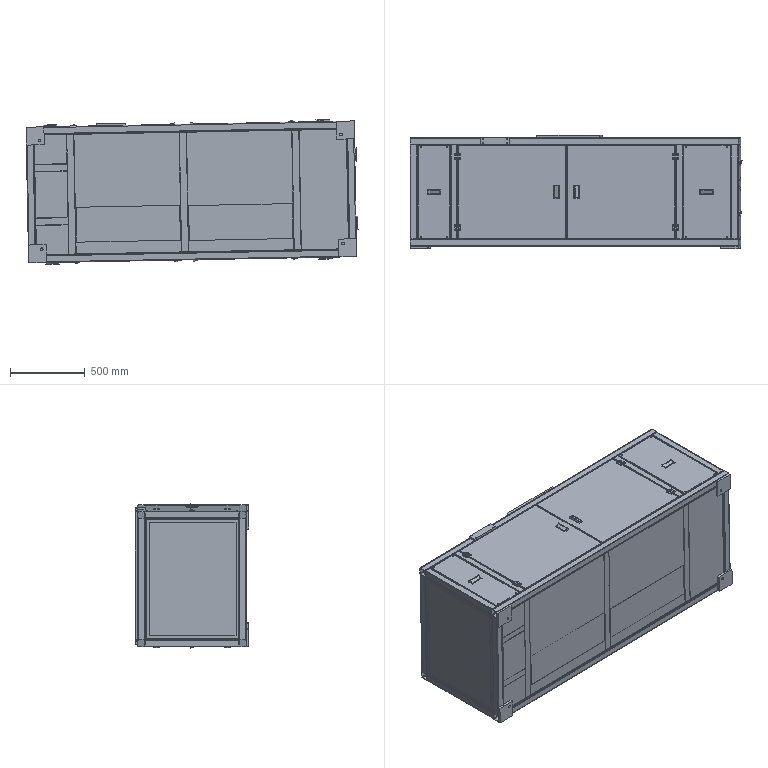Assembly | SolidWorks | mm | 44 component files | 133 solids | 3777 faces | box 2225.49 x 760 x 970.37 mm | volume 42957935 mm3 | plane 2257 | cylinder 1328 | cone 192 | commonest cylinder face diameters 6 x200 10 x144 7 x122 2 x120 5 x104 4.2 x100 4 x88 11 x72
Bill of materials:
01Frame | 1 | A3 Steel | Elongated rectangular open frame built from square-section members, with corner blocks, intermediate vertical posts and cross members, one long side covered by a flat panel, and an internal partition panel near one end.
02FrameEndPlate1 | 2 | A3 Steel | Rectangular tray-like cover plate with shallow turned-down edge flanges, one central rectangular cutout and four corner holes.
03FrameEndPlate2 | 2 | A3 Steel | Long, narrow rectangular cover plate with shallow turned-down edge flanges, one central rectangular cutout and four corner holes.
04FrameEndPlate3 | 2 | A3 Steel | Tall rectangular flat panel with a shallow edge return, two vertically aligned rectangular slots on the centerline and small holes near the four corners.
05FrameEndPlate4 | 1 | A3 Steel | Rectangular flat panel with a shallow edge return, two vertically aligned rectangular slots on the centerline and small holes near the four corners. It is wider than the similar slotted panel.
09Panel2 | 1 | A3 Steel | Flat rectangular plate with a large rectangular window that has rounded corners, plus many small holes in clusters above and below the window and along the edges.
11BottomDoor | 2 | A3 Steel | Large, nearly square flat panel with a shallow perimeter flange, one off-center rectangular slot near an edge and a few small holes near two corners.
12TopPostMountingPlateSpacer | 2 | A3 Steel | Solid rectangular bar or block with two round through-holes passing through its narrow side face.
13TopPostMountingPlate | 1 | A3 Steel | Thick rectangular plate with two parallel columns of evenly spaced round holes and four elongated slots near the corners.
15BrushPlateThickInnerFrameOneOutOfTwo | 1 | A3 Steel | Rectangular frame plate with rounded outer corners, a large central opening with stepped notches, small mounting holes around the perimeter, and stepped raised rails along the inner edges.
16MeshPlateOneOutOfTwo | 1 | A3 Steel | Thin flat sheet plate with rounded corners, four long parallel slots, four larger corner holes and several small edge holes.
17DustCollectionHopper | 2 | A3 Steel | Long formed sheet channel panel: a flat face with a top return flange and curled hook-shaped flanges at both ends.
22DragChainMountingPlate | 1 | A3 Steel | Long, slender straight channel with a C-shaped cross-section and rounded bends, with small holes near both ends and at mid-length.
23BottomDoor2 | 2 | A3 Steel | Large, thin, nearly square panel with shallow bent-down edge flanges, one rectangular through-cutout near one edge, and small holes near two corners.
40X40AluminumAlloyHinge | 8 | A3 Steel | Square flat plate with four through-holes, one near each corner, and a cylindrical (rounded) rib on the underside running across the plate.
93X35EmbeddedHandleSlot87X30.5 | 14 | A3 Steel | Elongated prismatic block with a wedge-shaped (sloped) top on a narrower rectangular base, with a shallow L-shaped groove or recess on the sloped face.
PowerDistributionCabinet | 1 | A3 Steel | Plain solid rectangular block (cuboid) with no visible holes, cutouts or other features.
Mates:
1. coincident | 15BrushPlateThickInnerFrameOneOutOfTwo-1 face at (111.137, -1638.022, 1897.203) dir (0, -1, 0) | 16MeshPlateOneOutOfTwo-1 face at (104.662, -1638.022, 2237.141) dir (0, 1, 0)
2. coincident | 09Panel2-1 face at (76.81, -1621.522, 1861.543) dir (0, 1, 0) | 15BrushPlateThickInnerFrameOneOutOfTwo-1 face at (368.947, -1621.522, 2277.182) dir (0, -1, 0)
3. coincident | 09Panel2-1 face at (77.095, -1621.522, 1846.545) dir (-0.01904, 0, 0.9998) | 15BrushPlateThickInnerFrameOneOutOfTwo-1 face at (77.095, -1621.522, 1846.545) dir (0.01904, 0, -0.9998)
4. coincident | 09Panel2-1 face at (61.812, -1621.522, 1861.257) dir (0.9998, 0, 0.01904) | 15BrushPlateThickInnerFrameOneOutOfTwo-1 face at (61.812, -1621.522, 1861.257) dir (-0.9998, 0, -0.01904)
5. coincident | 11BottomDoor-1 face at (-158.243, -1995.522, 2387.162) dir (-0.01904, 0, 0.9998) | 93X35EmbeddedHandleSlot87X30.5-18 face at (157.2, -2041.272, 2393.17) dir (0.01904, 0, -0.9998)
6. coincident | 11BottomDoor-1 edge at (124.706, -1952.022, 2392.551) dir (0, -1, 0) | 93X35EmbeddedHandleSlot87X30.5-18 face at (124.82, -1952.022, 2386.552) dir (-0.9998, 0, -0.01904)
7. coincident | 13TopPostMountingPlate-1 plane at (1160.151, -1828.022, 2090.216) dir (0.9998, 0, 0.01904) | 12TopPostMountingPlateSpacer-1 plane at (1158.199, -1865.522, 2192.697) dir (0.9998, 0, 0.01904)
8. coincident | 01Frame-1 face at (257.063, -1995.522, 2375.069) dir (-0.01904, 0, 0.9998) | 02FrameEndPlate1-1 face at (1146.901, -1995.522, 2392.018) dir (0.01904, 0, -0.9998)
9. coincident | 01Frame-1 face at (273.631, -1995.522, 1505.226) dir (0.01904, 0, -0.9998) | 02FrameEndPlate1-2 face at (1163.47, -1995.522, 1522.176) dir (-0.01904, 0, 0.9998)
10. concentric | 01Frame-1 face at (1025.995, -2297.522, 1519.557) dir (0.01904, 0, -0.9998) r 2.5 | 02FrameEndPlate1-2 face at (1026.376, -2297.522, 1499.561) dir (0.01904, 0, -0.9998) r 3.5
11. coincident | 01Frame-1 face at (257.063, -1995.522, 2375.069) dir (-0.01904, 0, 0.9998) | 03FrameEndPlate2-1 face at (-682.767, -1995.522, 2357.167) dir (0.01904, 0, -0.9998)
12. concentric | 01Frame-1 face at (-770.251, -1693.522, 2355.501) dir (-0.01904, 0, 0.9998) r 2.5 | 03FrameEndPlate2-1 face at (-770.632, -1693.522, 2375.497) dir (-0.01904, 0, 0.9998) r 3.5
13. concentric | 01Frame-1 face at (-595.283, -2297.522, 2358.833) dir (-0.01904, 0, 0.9998) r 2.5 | 03FrameEndPlate2-1 face at (-595.664, -2297.522, 2378.83) dir (-0.01904, 0, 0.9998) r 3.5
14. coincident | 01Frame-1 face at (273.631, -1995.522, 1505.226) dir (0.01904, 0, -0.9998) | 03FrameEndPlate2-2 face at (-666.198, -1995.522, 1487.325) dir (-0.01904, 0, 0.9998)
15. concentric | 01Frame-1 face at (-753.682, -2297.522, 1485.658) dir (0.01904, 0, -0.9998) r 2.5 | 03FrameEndPlate2-2 face at (-753.302, -2297.522, 1465.662) dir (0.01904, 0, -0.9998) r 3.5
16. concentric | 01Frame-1 face at (-578.714, -1693.522, 1488.991) dir (0.01904, 0, -0.9998) r 2.5 | 03FrameEndPlate2-2 edge at (-578.371, -1693.522, 1470.994) dir (-0.01904, 0, 0.9998) r 3.5
17. coincident | 01Frame-1 face at (1353.34, -1995.522, 1530.793) dir (0.9998, 0, 0.01904) | 04FrameEndPlate3-1 face at (1345.151, -1798.022, 1960.715) dir (-0.9998, 0, -0.01904)
18. concentric | 01Frame-1 edge at (1337.867, -1693.522, 2343.146) dir (0.9998, 0, 0.01904) r 2.5 | 04FrameEndPlate3-1 face at (1357.863, -1693.522, 2343.527) dir (0.9998, 0, 0.01904) r 3.5
19. concentric | 01Frame-1 face at (1352.436, -1902.522, 1578.285) dir (0.9998, 0, 0.01904) r 2.5 | 04FrameEndPlate3-1 face at (1372.432, -1902.522, 1578.666) dir (0.9998, 0, 0.01904) r 3.5
20. coincident | 01Frame-1 face at (1336.962, -1995.522, 2390.637) dir (0.9998, 0, 0.01904) | 05FrameEndPlate4-1 face at (1345.151, -2138.022, 1960.715) dir (-0.9998, 0, -0.01904)
21. concentric | 01Frame-1 face at (1352.436, -1979.522, 1578.285) dir (0.9998, 0, 0.01904) r 2.5 | 05FrameEndPlate4-1 face at (1372.432, -1979.522, 1578.666) dir (0.9998, 0, 0.01904) r 3.5
22. concentric | 01Frame-1 face at (1337.867, -2296.522, 2343.146) dir (0.9998, 0, 0.01904) r 2.5 | 05FrameEndPlate4-1 face at (1357.863, -2296.522, 2343.527) dir (0.9998, 0, 0.01904) r 3.5
23. coincident | 01Frame-1 face at (1348.722, -1630.522, 1510.702) dir (0, 1, 0) | 09Panel2-1 face at (225.259, -1630.522, 1944.385) dir (0, -1, 0)
24. coincident | 01Frame-1 face at (1331.487, -1675.522, 2415.538) dir (-0.01904, 0, 0.9998) | 09Panel2-1 face at (6.727, -1615.522, 2390.304) dir (-0.01904, 0, 0.9998)
25. coincident | 01Frame-1 face at (-787.414, -2310.522, 2075.123) dir (0, 1, 0) | PowerDistributionCabinet-1 face at (-592.497, -2310.522, 1923.808) dir (0, -1, 0)
26. coincident | 01Frame-1 face at (-842.262, -1655.522, 2329.124) dir (-0.9998, 0, -0.01904) | PowerDistributionCabinet-1 face at (-834.454, -1999.522, 1919.199) dir (-0.9998, 0, -0.01904)
27. distance | PowerDistributionCabinet-1 face at (-584.88, -1999.522, 1523.88) dir (0.01904, 0, -0.9998) | 01Frame-1 face at (-781.749, -1655.522, 1515.129) dir (-0.01904, 0, 0.9998)
28. coincident | 01Frame-1 face at (-528.176, -1655.522, 2380.115) dir (-0.01904, 0, 0.9998) | 11BottomDoor-1 face at (-158.243, -1995.522, 2387.162) dir (-0.01904, 0, 0.9998)
29. coincident | 01Frame-1 face at (273.536, -2347.522, 1510.226) dir (0, 1, 0) | 17DustCollectionHopper-1 face at (596.252, -2347.522, 1738.254) dir (0, -1, 0)
30. distance | 17DustCollectionHopper-1 face at (246.315, -2345.522, 1731.588) dir (-0.9998, 0, -0.01904) | 01Frame-1 face at (248.064, -2310.522, 1534.745) dir (0.9998, 0, 0.01904)
31. coincident | 01Frame-1 face at (273.536, -2347.522, 1510.226) dir (0, 1, 0) | 17DustCollectionHopper-3 face at (-157.672, -2347.522, 1727.053) dir (0, -1, 0)
32. distance | 17DustCollectionHopper-3 face at (192.265, -2345.522, 1733.718) dir (0.9998, 0, 0.01904) | 01Frame-1 face at (198.073, -2310.522, 1533.793) dir (-0.9998, 0, -0.01904)
33. coincident | 01Frame-1 face at (273.536, -1895.522, 1510.226) dir (0, 1, 0) | 12TopPostMountingPlateSpacer-1 face at (1158.199, -1895.522, 2192.697) dir (0, -1, 0)
34. distance | 13TopPostMountingPlate-1 plane at (1160.151, -1828.022, 2090.216) dir (0.01904, 0, -0.9998) | 01Frame-1 face at (1279.296, -1895.522, 2267.517) dir (-0.01904, 0, 0.9998)
35. coincident | 02FrameEndPlate1-1 face at (1146.52, -1995.522, 2412.014) dir (-0.01904, 0, 0.9998) | 93X35EmbeddedHandleSlot87X30.5-4 face at (1192.262, -1978.272, 2412.886) dir (0.01904, 0, -0.9998)
36. coincident | 02FrameEndPlate1-1 face at (1190.393, -2010.772, 2392.846) dir (-0.9998, 0, -0.01904) | 93X35EmbeddedHandleSlot87X30.5-4 face at (1190.127, -1980.272, 2406.844) dir (0.9998, 0, 0.01904)
37. coincident | 02FrameEndPlate1-1 edge at (1190.013, -1980.272, 2412.843) dir (-0.9998, 0, -0.01904) | 93X35EmbeddedHandleSlot87X30.5-4 face at (1103.143, -1980.272, 2405.187) dir (0, 1, 0)
38. coincident | 02FrameEndPlate1-2 face at (1163.851, -1995.522, 1502.179) dir (0.01904, 0, -0.9998) | 93X35EmbeddedHandleSlot87X30.5-3 face at (1118.109, -1978.272, 1501.308) dir (-0.01904, 0, 0.9998)
39. coincident | 02FrameEndPlate1-2 face at (1119.978, -2010.772, 1521.347) dir (0.9998, 0, 0.01904) | 93X35EmbeddedHandleSlot87X30.5-3 face at (1120.244, -1980.272, 1507.35) dir (-0.9998, 0, -0.01904)
40. coincident | 02FrameEndPlate1-2 face at (1206.962, -1980.272, 1523.004) dir (0, -1, 0) | 93X35EmbeddedHandleSlot87X30.5-3 face at (1207.229, -1980.272, 1509.007) dir (0, 1, 0)
41. coincident | 03FrameEndPlate2-1 face at (-683.148, -1995.522, 2377.163) dir (-0.01904, 0, 0.9998) | 93X35EmbeddedHandleSlot87X30.5-1 face at (-637.406, -1978.272, 2378.035) dir (0.01904, 0, -0.9998)
42. coincident | 03FrameEndPlate2-1 face at (-726.259, -1980.272, 2356.339) dir (0, -1, 0) | 93X35EmbeddedHandleSlot87X30.5-1 face at (-726.526, -1980.272, 2370.336) dir (0, 1, 0)
43. distance | 93X35EmbeddedHandleSlot87X30.5-1 face at (-726.526, -1980.272, 2370.336) dir (-0.9998, 0, -0.01904) | 03FrameEndPlate2-1 face at (-726.259, -2010.772, 2356.339) dir (0.9998, 0, 0.01904)
44. coincident | 03FrameEndPlate2-2 face at (-665.817, -1995.522, 1467.328) dir (0.01904, 0, -0.9998) | 93X35EmbeddedHandleSlot87X30.5-2 face at (-711.559, -1978.272, 1466.457) dir (-0.01904, 0, 0.9998)
45. coincident | 03FrameEndPlate2-2 edge at (-709.31, -2010.772, 1466.5) dir (0, 1, 0) | 93X35EmbeddedHandleSlot87X30.5-2 face at (-709.424, -1980.272, 1472.499) dir (-0.9998, 0, -0.01904)
46. coincident | 03FrameEndPlate2-2 face at (-622.706, -1980.272, 1488.153) dir (0, -1, 0) | 93X35EmbeddedHandleSlot87X30.5-2 face at (-622.44, -1980.272, 1474.156) dir (0, 1, 0)
47. coincident | 04FrameEndPlate3-1 face at (1365.147, -1798.022, 1961.096) dir (0.9998, 0, 0.01904) | 93X35EmbeddedHandleSlot87X30.5-5 face at (1361.639, -1780.772, 2145.313) dir (-0.9998, 0, -0.01904)
48. coincident | 04FrameEndPlate3-1 face at (1339.942, -1782.772, 2234.166) dir (0.01904, 0, -0.9998) | 93X35EmbeddedHandleSlot87X30.5-5 face at (1353.94, -1782.772, 2234.432) dir (-0.01904, 0, 0.9998)
49. coincident | 04FrameEndPlate3-1 edge at (1359.596, -1813.272, 2147.524) dir (-0.01904, 0, 0.9998) | 93X35EmbeddedHandleSlot87X30.5-5 face at (1353.94, -1813.272, 2234.432) dir (0, -1, 0)
50. coincident | 05FrameEndPlate4-1 face at (1341.599, -2122.772, 2147.182) dir (-0.01904, 0, 0.9998) | 93X35EmbeddedHandleSlot87X30.5-14 face at (1355.597, -2122.772, 2147.448) dir (0.01904, 0, -0.9998)
51. coincident | 05FrameEndPlate4-1 face at (1341.599, -2153.272, 2147.182) dir (0, 1, 0) | 93X35EmbeddedHandleSlot87X30.5-14 face at (1353.94, -2153.272, 2234.432) dir (0, -1, 0)
52. coincident | 05FrameEndPlate4-1 face at (1365.147, -2138.022, 1961.096) dir (0.9998, 0, 0.01904) | 93X35EmbeddedHandleSlot87X30.5-14 face at (1361.639, -2120.772, 2145.313) dir (-0.9998, 0, -0.01904)
53. coincident | 01Frame-1 face at (-528.176, -1655.522, 2380.115) dir (-0.01904, 0, 0.9998) | 40X40AluminumAlloyHinge-7 face at (-523.177, -1758.022, 2380.21) dir (0.01904, 0, -0.9998)
54. concentric | 01Frame-1 face at (-535.674, -1745.522, 2379.972) dir (-0.01904, 0, 0.9998) r 2.1 | 40X40AluminumAlloyHinge-7 face at (-535.77, -1745.522, 2384.972) dir (-0.01904, 0, 0.9998) r 2.75
55. concentric | 01Frame-1 face at (-535.674, -1770.522, 2379.972) dir (-0.01904, 0, 0.9998) r 2.1 | 40X40AluminumAlloyHinge-7 face at (-535.77, -1770.522, 2384.972) dir (-0.01904, 0, 0.9998) r 2.75
56. concentric | 11BottomDoor-1 face at (-510.679, -1770.522, 2380.449) dir (-0.01904, 0, 0.9998) r 2.1 | 40X40AluminumAlloyHinge-7 face at (-510.774, -1770.522, 2385.448) dir (-0.01904, 0, 0.9998) r 2.75
57. concentric | 11BottomDoor-1 face at (-510.679, -1745.522, 2380.449) dir (-0.01904, 0, 0.9998) r 2.1 | 40X40AluminumAlloyHinge-7 face at (-510.774, -1745.522, 2385.448) dir (-0.01904, 0, 0.9998) r 2.75
58. coincident | 13TopPostMountingPlate-1 face at (1160.151, -1835.522, 2090.216) dir (0, -1, 0) | 12TopPostMountingPlateSpacer-1 face at (1158.199, -1835.522, 2192.697) dir (0, 1, 0)
59. coincident | 15BrushPlateThickInnerFrameOneOutOfTwo-1 face at (101.139, -1638.022, 1897.012) dir (0.9998, 0, 0.01904) | 16MeshPlateOneOutOfTwo-1 face at (101.139, -1638.022, 1897.012) dir (-0.9998, 0, -0.01904)
60. coincident | 15BrushPlateThickInnerFrameOneOutOfTwo-1 face at (104.471, -1638.022, 2247.139) dir (0.01904, 0, -0.9998) | 16MeshPlateOneOutOfTwo-1 face at (334.43, -1638.022, 2251.52) dir (-0.01904, 0, 0.9998)
61. concentric | 01Frame-1 face at (1218.188, -1895.522, 2193.84) dir (0, 1, 0) r 3.4 | 12TopPostMountingPlateSpacer-1 face at (1218.188, -1835.522, 2193.84) dir (0, 1, 0) r 7.5
62. coincident | 01Frame-1 face at (248.064, -2310.522, 1534.745) dir (0, 1, 0) | 22DragChainMountingPlate-1 face at (988.463, -2310.522, 2308.486) dir (0, -1, 0)
63. concentric | 01Frame-1 edge at (-533.461, -2310.522, 2289.998) dir (0, 1, 0) r 1.65 | 22DragChainMountingPlate-1 edge at (-533.461, -2308.522, 2289.998) dir (0, 1, 0) r 4.3
64. concentric | 01Frame-1 face at (975.789, -2310.522, 2343.751) dir (0, 1, 0) r 1.65 | 22DragChainMountingPlate-1 edge at (975.789, -2308.522, 2343.751) dir (0, 1, 0) r 4.3
65. distance | 17DustCollectionHopper-3 face at (-155.386, -2345.522, 1607.075) dir (0.01904, 0, -0.9998) | 01Frame-1 face at (1347.865, -2315.522, 1555.694) dir (-0.01904, 0, 0.9998)
66. concentric | 01Frame-1 edge at (1009.426, -1693.522, 2389.399) dir (-0.01904, 0, 0.9998) r 2.5 | 02FrameEndPlate1-1 face at (1009.045, -1693.522, 2409.396) dir (-0.01904, 0, 0.9998) r 3.5
67. concentric | 01Frame-1 face at (1284.376, -2297.522, 2394.637) dir (-0.01904, 0, 0.9998) r 2.5 | 02FrameEndPlate1-1 face at (1283.995, -2297.522, 2414.633) dir (-0.01904, 0, 0.9998) r 3.5
68. concentric | 01Frame-1 face at (1300.945, -1693.522, 1524.794) dir (0.01904, 0, -0.9998) r 2.5 | 02FrameEndPlate1-2 face at (1301.326, -1693.522, 1504.798) dir (0.01904, 0, -0.9998) r 3.5
69. coincident | 01Frame-1 face at (981.55, -1655.522, 2408.872) dir (-0.01904, 0, 0.9998) | 23BottomDoor2-1 face at (571.625, -1995.522, 2401.064) dir (-0.01904, 0, 0.9998)
70. concentric | 40X40AluminumAlloyHinge-5 edge at (923.966, -1745.522, 2412.776) dir (-0.01904, 0, 0.9998) r 5.6 | 23BottomDoor2-1 edge at (924.061, -1745.522, 2407.777) dir (-0.01904, 0, 0.9998) r 2.1
71. concentric | 40X40AluminumAlloyHinge-6 face at (923.966, -2220.522, 2412.776) dir (-0.01904, 0, 0.9998) r 2.75 | 23BottomDoor2-1 face at (924.061, -2220.522, 2407.777) dir (-0.01904, 0, 0.9998) r 2.1
72. distance | 11BottomDoor-1 face at (155.581, -2039.022, 2373.136) dir (0, 1, 0) | 93X35EmbeddedHandleSlot87X30.5-18 face at (139.953, -2041.272, 2392.842) dir (0, -1, 0)